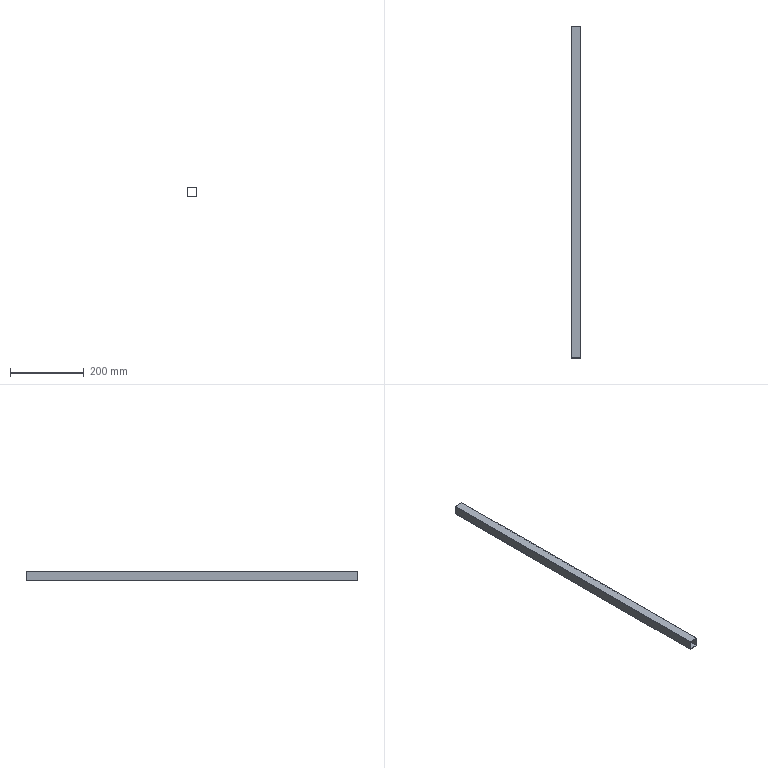Component | SolidWorks | AwningSupportRod-5 | 1 solid | 10 faces | box 25 x 898.5 x 25 mm | volume 126688 mm3 | plane 10
build123d program:
from build123d import *

# Parameters (mm, degrees)
SKETCH1_W           = 25
SKETCH1_H           = 25
SKETCH1_W_2         = 22
SKETCH1_H_2         = 22
BOSS_EXTRUDE1_DEPTH = 898.5


with BuildPart() as part:
    # Sketch1 → Boss-Extrude1 (new body)
    with BuildSketch(Plane(origin=(0, 0, 0), x_dir=(1, 0, 0), z_dir=(0, 1, 0))):
        Rectangle(SKETCH1_W, SKETCH1_H)
        Rectangle(SKETCH1_W_2, SKETCH1_H_2, mode=Mode.SUBTRACT)
    extrude(amount=BOSS_EXTRUDE1_DEPTH)


solid = part.part

# Placed as in the assembly
solid = solid.moved(Location((257.5, 800, -257.5), (0, 0, 0)))
STEP:
#1=COLOUR_RGB('',0.7922,0.8196,0.9333);
#2=FILL_AREA_STYLE_COLOUR('',#1);
#3=FILL_AREA_STYLE('',(#2));
#4=SURFACE_STYLE_FILL_AREA(#3);
#5=SURFACE_SIDE_STYLE('',(#4));
#6=SURFACE_STYLE_USAGE(.BOTH.,#5);
#7=PRESENTATION_STYLE_ASSIGNMENT((#6));
#8=CARTESIAN_POINT('',(9.646,66.87,-10.63));
#9=VERTEX_POINT('',#8);
#10=CARTESIAN_POINT('',(9.646,66.87,-9.646));
#11=VERTEX_POINT('',#10);
#12=CARTESIAN_POINT('',(9.646,66.87,-9.646));
#13=DIRECTION('',(0.,0.,1.));
#14=VECTOR('',#13,39.37);
#15=LINE('',#12,#14);
#16=EDGE_CURVE('',#9,#11,#15,.T.);
#17=ORIENTED_EDGE('',*,*,#16,.T.);
#18=CARTESIAN_POINT('',(10.63,66.87,-9.646));
#19=VERTEX_POINT('',#18);
#20=CARTESIAN_POINT('',(10.63,66.87,-9.646));
#21=DIRECTION('',(1.,0.,-0.));
#22=VECTOR('',#21,39.37);
#23=LINE('',#20,#22);
#24=EDGE_CURVE('',#11,#19,#23,.T.);
#25=ORIENTED_EDGE('',*,*,#24,.T.);
#26=CARTESIAN_POINT('',(10.63,66.87,-10.63));
#27=VERTEX_POINT('',#26);
#28=CARTESIAN_POINT('',(10.63,66.87,-9.646));
#29=DIRECTION('',(0.,-0.,-1.));
#30=VECTOR('',#29,39.37);
#31=LINE('',#28,#30);
#32=EDGE_CURVE('',#19,#27,#31,.T.);
#33=ORIENTED_EDGE('',*,*,#32,.T.);
#34=CARTESIAN_POINT('',(10.63,66.87,-10.63));
#35=DIRECTION('',(-1.,-0.,0.));
#36=VECTOR('',#35,39.37);
#37=LINE('',#34,#36);
#38=EDGE_CURVE('',#27,#9,#37,.T.);
#39=ORIENTED_EDGE('',*,*,#38,.T.);
#40=EDGE_LOOP('',(#17,#25,#33,#39));
#41=FACE_OUTER_BOUND('',#40,.T.);
#42=CARTESIAN_POINT('',(9.705,66.87,-9.705));
#43=VERTEX_POINT('',#42);
#44=CARTESIAN_POINT('',(10.571,66.87,-9.705));
#45=VERTEX_POINT('',#44);
#46=CARTESIAN_POINT('',(10.571,66.87,-9.705));
#47=DIRECTION('',(1.,0.,-0.));
#48=VECTOR('',#47,39.37);
#49=LINE('',#46,#48);
#50=EDGE_CURVE('',#43,#45,#49,.T.);
#51=ORIENTED_EDGE('',*,*,#50,.F.);
#52=CARTESIAN_POINT('',(9.705,66.87,-10.571));
#53=VERTEX_POINT('',#52);
#54=CARTESIAN_POINT('',(9.705,66.87,-9.705));
#55=DIRECTION('',(0.,0.,1.));
#56=VECTOR('',#55,39.37);
#57=LINE('',#54,#56);
#58=EDGE_CURVE('',#53,#43,#57,.T.);
#59=ORIENTED_EDGE('',*,*,#58,.F.);
#60=CARTESIAN_POINT('',(10.571,66.87,-10.571));
#61=VERTEX_POINT('',#60);
#62=CARTESIAN_POINT('',(10.571,66.87,-10.571));
#63=DIRECTION('',(-1.,-0.,0.));
#64=VECTOR('',#63,39.37);
#65=LINE('',#62,#64);
#66=EDGE_CURVE('',#61,#53,#65,.T.);
#67=ORIENTED_EDGE('',*,*,#66,.F.);
#68=CARTESIAN_POINT('',(10.571,66.87,-9.705));
#69=DIRECTION('',(0.,-0.,-1.));
#70=VECTOR('',#69,39.37);
#71=LINE('',#68,#70);
#72=EDGE_CURVE('',#45,#61,#71,.T.);
#73=ORIENTED_EDGE('',*,*,#72,.F.);
#74=EDGE_LOOP('',(#51,#59,#67,#73));
#75=FACE_BOUND('',#74,.T.);
#76=CARTESIAN_POINT('',(10.138,66.87,-10.138));
#77=DIRECTION('',(-0.,1.,-0.));
#78=DIRECTION('',(0.,-0.,-1.));
#79=AXIS2_PLACEMENT_3D('',#76,#77,#78);
#80=PLANE('',#79);
#81=ADVANCED_FACE('',(#41,#75),#80,.T.);
#82=CARTESIAN_POINT('',(9.646,31.496,-10.63));
#83=VERTEX_POINT('',#82);
#84=CARTESIAN_POINT('',(9.646,31.496,-9.646));
#85=VERTEX_POINT('',#84);
#86=CARTESIAN_POINT('',(9.646,31.496,-9.646));
#87=DIRECTION('',(0.,0.,1.));
#88=VECTOR('',#87,39.37);
#89=LINE('',#86,#88);
#90=EDGE_CURVE('',#83,#85,#89,.T.);
#91=ORIENTED_EDGE('',*,*,#90,.F.);
#92=CARTESIAN_POINT('',(10.63,31.496,-10.63));
#93=VERTEX_POINT('',#92);
#94=CARTESIAN_POINT('',(10.63,31.496,-10.63));
#95=DIRECTION('',(-1.,-0.,0.));
#96=VECTOR('',#95,39.37);
#97=LINE('',#94,#96);
#98=EDGE_CURVE('',#93,#83,#97,.T.);
#99=ORIENTED_EDGE('',*,*,#98,.F.);
#100=CARTESIAN_POINT('',(10.63,31.496,-9.646));
#101=VERTEX_POINT('',#100);
#102=CARTESIAN_POINT('',(10.63,31.496,-9.646));
#103=DIRECTION('',(0.,-0.,-1.));
#104=VECTOR('',#103,39.37);
#105=LINE('',#102,#104);
#106=EDGE_CURVE('',#101,#93,#105,.T.);
#107=ORIENTED_EDGE('',*,*,#106,.F.);
#108=CARTESIAN_POINT('',(10.63,31.496,-9.646));
#109=DIRECTION('',(1.,0.,-0.));
#110=VECTOR('',#109,39.37);
#111=LINE('',#108,#110);
#112=EDGE_CURVE('',#85,#101,#111,.T.);
#113=ORIENTED_EDGE('',*,*,#112,.F.);
#114=EDGE_LOOP('',(#91,#99,#107,#113));
#115=FACE_OUTER_BOUND('',#114,.T.);
#116=CARTESIAN_POINT('',(9.705,31.496,-10.571));
#117=VERTEX_POINT('',#116);
#118=CARTESIAN_POINT('',(9.705,31.496,-9.705));
#119=VERTEX_POINT('',#118);
#120=CARTESIAN_POINT('',(9.705,31.496,-9.705));
#121=DIRECTION('',(0.,0.,1.));
#122=VECTOR('',#121,39.37);
#123=LINE('',#120,#122);
#124=EDGE_CURVE('',#117,#119,#123,.T.);
#125=ORIENTED_EDGE('',*,*,#124,.T.);
#126=CARTESIAN_POINT('',(10.571,31.496,-9.705));
#127=VERTEX_POINT('',#126);
#128=CARTESIAN_POINT('',(10.571,31.496,-9.705));
#129=DIRECTION('',(1.,0.,-0.));
#130=VECTOR('',#129,39.37);
#131=LINE('',#128,#130);
#132=EDGE_CURVE('',#119,#127,#131,.T.);
#133=ORIENTED_EDGE('',*,*,#132,.T.);
#134=CARTESIAN_POINT('',(10.571,31.496,-10.571));
#135=VERTEX_POINT('',#134);
#136=CARTESIAN_POINT('',(10.571,31.496,-9.705));
#137=DIRECTION('',(0.,-0.,-1.));
#138=VECTOR('',#137,39.37);
#139=LINE('',#136,#138);
#140=EDGE_CURVE('',#127,#135,#139,.T.);
#141=ORIENTED_EDGE('',*,*,#140,.T.);
#142=CARTESIAN_POINT('',(10.571,31.496,-10.571));
#143=DIRECTION('',(-1.,-0.,0.));
#144=VECTOR('',#143,39.37);
#145=LINE('',#142,#144);
#146=EDGE_CURVE('',#135,#117,#145,.T.);
#147=ORIENTED_EDGE('',*,*,#146,.T.);
#148=EDGE_LOOP('',(#125,#133,#141,#147));
#149=FACE_BOUND('',#148,.T.);
#150=CARTESIAN_POINT('',(10.138,31.496,-10.138));
#151=DIRECTION('',(-0.,1.,-0.));
#152=DIRECTION('',(0.,-0.,-1.));
#153=AXIS2_PLACEMENT_3D('',#150,#151,#152);
#154=PLANE('',#153);
#155=ADVANCED_FACE('',(#115,#149),#154,.F.);
#156=ORIENTED_EDGE('',*,*,#90,.T.);
#157=CARTESIAN_POINT('',(9.646,66.87,-9.646));
#158=DIRECTION('',(0.,-1.,0.));
#159=VECTOR('',#158,39.37);
#160=LINE('',#157,#159);
#161=EDGE_CURVE('',#11,#85,#160,.T.);
#162=ORIENTED_EDGE('',*,*,#161,.F.);
#163=ORIENTED_EDGE('',*,*,#16,.F.);
#164=CARTESIAN_POINT('',(9.646,66.87,-10.63));
#165=DIRECTION('',(0.,-1.,0.));
#166=VECTOR('',#165,39.37);
#167=LINE('',#164,#166);
#168=EDGE_CURVE('',#9,#83,#167,.T.);
#169=ORIENTED_EDGE('',*,*,#168,.T.);
#170=EDGE_LOOP('',(#156,#162,#163,#169));
#171=FACE_OUTER_BOUND('',#170,.T.);
#172=CARTESIAN_POINT('',(9.646,66.87,-9.646));
#173=DIRECTION('',(1.,0.,-0.));
#174=DIRECTION('',(0.,-0.,-1.));
#175=AXIS2_PLACEMENT_3D('',#172,#173,#174);
#176=PLANE('',#175);
#177=ADVANCED_FACE('',(#171),#176,.F.);
#178=ORIENTED_EDGE('',*,*,#112,.T.);
#179=CARTESIAN_POINT('',(10.63,66.87,-9.646));
#180=DIRECTION('',(0.,-1.,0.));
#181=VECTOR('',#180,39.37);
#182=LINE('',#179,#181);
#183=EDGE_CURVE('',#19,#101,#182,.T.);
#184=ORIENTED_EDGE('',*,*,#183,.F.);
#185=ORIENTED_EDGE('',*,*,#24,.F.);
#186=ORIENTED_EDGE('',*,*,#161,.T.);
#187=EDGE_LOOP('',(#178,#184,#185,#186));
#188=FACE_OUTER_BOUND('',#187,.T.);
#189=CARTESIAN_POINT('',(10.63,66.87,-9.646));
#190=DIRECTION('',(-0.,-0.,-1.));
#191=DIRECTION('',(-1.,-0.,0.));
#192=AXIS2_PLACEMENT_3D('',#189,#190,#191);
#193=PLANE('',#192);
#194=ADVANCED_FACE('',(#188),#193,.F.);
#195=ORIENTED_EDGE('',*,*,#106,.T.);
#196=CARTESIAN_POINT('',(10.63,66.87,-10.63));
#197=DIRECTION('',(0.,-1.,0.));
#198=VECTOR('',#197,39.37);
#199=LINE('',#196,#198);
#200=EDGE_CURVE('',#27,#93,#199,.T.);
#201=ORIENTED_EDGE('',*,*,#200,.F.);
#202=ORIENTED_EDGE('',*,*,#32,.F.);
#203=ORIENTED_EDGE('',*,*,#183,.T.);
#204=EDGE_LOOP('',(#195,#201,#202,#203));
#205=FACE_OUTER_BOUND('',#204,.T.);
#206=CARTESIAN_POINT('',(10.63,66.87,-9.646));
#207=DIRECTION('',(-1.,-0.,0.));
#208=DIRECTION('',(0.,0.,1.));
#209=AXIS2_PLACEMENT_3D('',#206,#207,#208);
#210=PLANE('',#209);
#211=ADVANCED_FACE('',(#205),#210,.F.);
#212=ORIENTED_EDGE('',*,*,#98,.T.);
#213=ORIENTED_EDGE('',*,*,#168,.F.);
#214=ORIENTED_EDGE('',*,*,#38,.F.);
#215=ORIENTED_EDGE('',*,*,#200,.T.);
#216=EDGE_LOOP('',(#212,#213,#214,#215));
#217=FACE_OUTER_BOUND('',#216,.T.);
#218=CARTESIAN_POINT('',(10.63,66.87,-10.63));
#219=DIRECTION('',(0.,0.,1.));
#220=DIRECTION('',(1.,0.,-0.));
#221=AXIS2_PLACEMENT_3D('',#218,#219,#220);
#222=PLANE('',#221);
#223=ADVANCED_FACE('',(#217),#222,.F.);
#224=ORIENTED_EDGE('',*,*,#124,.F.);
#225=CARTESIAN_POINT('',(9.705,66.87,-10.571));
#226=DIRECTION('',(0.,-1.,0.));
#227=VECTOR('',#226,39.37);
#228=LINE('',#225,#227);
#229=EDGE_CURVE('',#53,#117,#228,.T.);
#230=ORIENTED_EDGE('',*,*,#229,.F.);
#231=ORIENTED_EDGE('',*,*,#58,.T.);
#232=CARTESIAN_POINT('',(9.705,66.87,-9.705));
#233=DIRECTION('',(0.,-1.,0.));
#234=VECTOR('',#233,39.37);
#235=LINE('',#232,#234);
#236=EDGE_CURVE('',#43,#119,#235,.T.);
#237=ORIENTED_EDGE('',*,*,#236,.T.);
#238=EDGE_LOOP('',(#224,#230,#231,#237));
#239=FACE_OUTER_BOUND('',#238,.T.);
#240=CARTESIAN_POINT('',(9.705,66.87,-9.705));
#241=DIRECTION('',(1.,0.,-0.));
#242=DIRECTION('',(0.,-0.,-1.));
#243=AXIS2_PLACEMENT_3D('',#240,#241,#242);
#244=PLANE('',#243);
#245=ADVANCED_FACE('',(#239),#244,.T.);
#246=ORIENTED_EDGE('',*,*,#132,.F.);
#247=ORIENTED_EDGE('',*,*,#236,.F.);
#248=ORIENTED_EDGE('',*,*,#50,.T.);
#249=CARTESIAN_POINT('',(10.571,66.87,-9.705));
#250=DIRECTION('',(0.,-1.,0.));
#251=VECTOR('',#250,39.37);
#252=LINE('',#249,#251);
#253=EDGE_CURVE('',#45,#127,#252,.T.);
#254=ORIENTED_EDGE('',*,*,#253,.T.);
#255=EDGE_LOOP('',(#246,#247,#248,#254));
#256=FACE_OUTER_BOUND('',#255,.T.);
#257=CARTESIAN_POINT('',(10.571,66.87,-9.705));
#258=DIRECTION('',(-0.,-0.,-1.));
#259=DIRECTION('',(-1.,-0.,0.));
#260=AXIS2_PLACEMENT_3D('',#257,#258,#259);
#261=PLANE('',#260);
#262=ADVANCED_FACE('',(#256),#261,.T.);
#263=ORIENTED_EDGE('',*,*,#140,.F.);
#264=ORIENTED_EDGE('',*,*,#253,.F.);
#265=ORIENTED_EDGE('',*,*,#72,.T.);
#266=CARTESIAN_POINT('',(10.571,66.87,-10.571));
#267=DIRECTION('',(0.,-1.,0.));
#268=VECTOR('',#267,39.37);
#269=LINE('',#266,#268);
#270=EDGE_CURVE('',#61,#135,#269,.T.);
#271=ORIENTED_EDGE('',*,*,#270,.T.);
#272=EDGE_LOOP('',(#263,#264,#265,#271));
#273=FACE_OUTER_BOUND('',#272,.T.);
#274=CARTESIAN_POINT('',(10.571,66.87,-9.705));
#275=DIRECTION('',(-1.,-0.,0.));
#276=DIRECTION('',(0.,0.,1.));
#277=AXIS2_PLACEMENT_3D('',#274,#275,#276);
#278=PLANE('',#277);
#279=ADVANCED_FACE('',(#273),#278,.T.);
#280=ORIENTED_EDGE('',*,*,#146,.F.);
#281=ORIENTED_EDGE('',*,*,#270,.F.);
#282=ORIENTED_EDGE('',*,*,#66,.T.);
#283=ORIENTED_EDGE('',*,*,#229,.T.);
#284=EDGE_LOOP('',(#280,#281,#282,#283));
#285=FACE_OUTER_BOUND('',#284,.T.);
#286=CARTESIAN_POINT('',(10.571,66.87,-10.571));
#287=DIRECTION('',(0.,0.,1.));
#288=DIRECTION('',(1.,0.,-0.));
#289=AXIS2_PLACEMENT_3D('',#286,#287,#288);
#290=PLANE('',#289);
#291=ADVANCED_FACE('',(#285),#290,.T.);
#292=CLOSED_SHELL('',(#81,#155,#177,#194,#211,#223,#245,#262,#279,#291));
#293=MANIFOLD_SOLID_BREP('',#292);
#294=STYLED_ITEM('',(#7),#293);
#295=PRESENTATION_LAYER_ASSIGNMENT('','',(#294));
#296=(LENGTH_UNIT()NAMED_UNIT(*)SI_UNIT($,.METRE.));
#297=LENGTH_MEASURE_WITH_UNIT(LENGTH_MEASURE(0.0254),#296);
#298=DIMENSIONAL_EXPONENTS(1.,0.,0.,0.,0.,0.,0.);
#299=(CONVERSION_BASED_UNIT('',#297)LENGTH_UNIT()NAMED_UNIT(#298));
#300=UNCERTAINTY_MEASURE_WITH_UNIT(LENGTH_MEASURE(0.00001),#299,'','');
#301=(NAMED_UNIT(*)PLANE_ANGLE_UNIT()SI_UNIT($,.RADIAN.));
#302=(NAMED_UNIT(*)SI_UNIT($,.STERADIAN.)SOLID_ANGLE_UNIT());
#303=(GEOMETRIC_REPRESENTATION_CONTEXT(3)GLOBAL_UNCERTAINTY_ASSIGNED_CONTEXT((#300))GLOBAL_UNIT_ASSIGNED_CONTEXT((#299,#301,#302))REPRESENTATION_CONTEXT('',''));
#304=MECHANICAL_DESIGN_GEOMETRIC_PRESENTATION_REPRESENTATION('',(#294),#303);
#305=CARTESIAN_POINT('',(0.,0.,0.));
#306=DIRECTION('',(0.,0.,1.));
#307=DIRECTION('',(1.,0.,0.));
#308=AXIS2_PLACEMENT_3D('',#305,#306,#307);
#309=(LENGTH_UNIT()NAMED_UNIT(*)SI_UNIT($,.METRE.));
#310=LENGTH_MEASURE_WITH_UNIT(LENGTH_MEASURE(0.0254),#309);
#311=DIMENSIONAL_EXPONENTS(1.,0.,0.,0.,0.,0.,0.);
#312=(CONVERSION_BASED_UNIT('',#310)LENGTH_UNIT()NAMED_UNIT(#311));
#313=UNCERTAINTY_MEASURE_WITH_UNIT(LENGTH_MEASURE(0.00001),#312,'','');
#314=(NAMED_UNIT(*)PLANE_ANGLE_UNIT()SI_UNIT($,.RADIAN.));
#315=(NAMED_UNIT(*)SI_UNIT($,.STERADIAN.)SOLID_ANGLE_UNIT());
#316=(GEOMETRIC_REPRESENTATION_CONTEXT(3)GLOBAL_UNCERTAINTY_ASSIGNED_CONTEXT((#313))GLOBAL_UNIT_ASSIGNED_CONTEXT((#312,#314,#315))REPRESENTATION_CONTEXT('',''));
#317=ADVANCED_BREP_SHAPE_REPRESENTATION('',(#293,#308),#316);